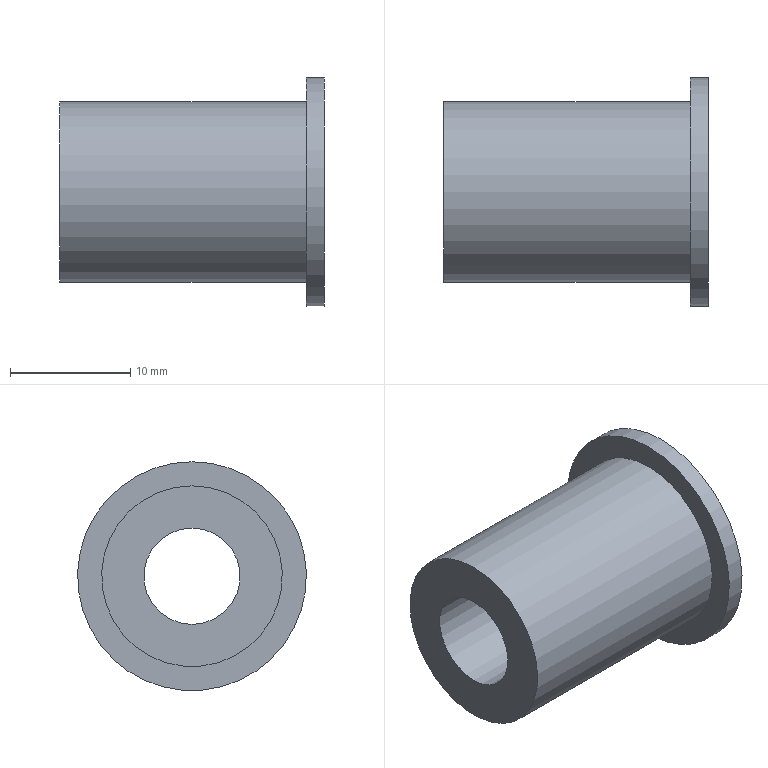Component | NX | HANDLE_BUSHING_2 | 1 solid | 6 faces | box 22 x 19 x 19 mm | volume 2942 mm3 | plane 3 | cylinder 3 | commonest cylinder face diameters 15 x1 19 x1 8 x1
STEP:
#1=CARTESIAN_POINT('',(0.,0.,0.));
#2=DIRECTION('',(0.,0.,1.));
#3=DIRECTION('',(1.,0.,0.));
#4=AXIS2_PLACEMENT_3D('',#1,#2,#3);
#5=CARTESIAN_POINT('',(184.037,-19.732,75.));
#6=VERTEX_POINT('',#5);
#7=CARTESIAN_POINT('',(184.037,-19.732,79.));
#8=DIRECTION('',(1.,0.,0.));
#9=DIRECTION('',(0.,0.,-1.));
#10=AXIS2_PLACEMENT_3D('',#7,#8,#9);
#11=CIRCLE('',#10,4.);
#12=CARTESIAN_POINT('',(184.037,-19.732,79.));
#13=DIRECTION('',(-1.,0.,0.));
#14=DIRECTION('',(0.,0.,1.));
#15=AXIS2_PLACEMENT_3D('',#12,#13,#14);
#16=PLANE('',#15);
#17=CARTESIAN_POINT('',(-4.,0.));
#18=CARTESIAN_POINT('',(-4.,6.928));
#19=CARTESIAN_POINT('',(2.,3.464));
#20=CARTESIAN_POINT('',(8.,0.));
#21=CARTESIAN_POINT('',(2.,-3.464));
#22=CARTESIAN_POINT('',(-4.,-6.928));
#23=CARTESIAN_POINT('',(-4.,0.));
#24=(BOUNDED_CURVE()B_SPLINE_CURVE(2,(#17,#18,#19,#20,#21,#22,#23),.UNSPECIFIED.,.T.,.F.)B_SPLINE_CURVE_WITH_KNOTS((1,2,2,2,2,1),(-2.094,0.,2.094,4.189,6.283,8.378),.UNSPECIFIED.)CURVE()GEOMETRIC_REPRESENTATION_ITEM()RATIONAL_B_SPLINE_CURVE((1.,0.5,1.,0.5,1.,0.5,1.))REPRESENTATION_ITEM(''));
#25=(GEOMETRIC_REPRESENTATION_CONTEXT(2)PARAMETRIC_REPRESENTATION_CONTEXT()REPRESENTATION_CONTEXT('',''));
#26=DEFINITIONAL_REPRESENTATION('',(#24),#25);
#27=PCURVE('',#16,#26);
#28=CARTESIAN_POINT('',(184.037,-19.732,79.));
#29=DIRECTION('',(1.,0.,0.));
#30=DIRECTION('',(0.,0.,-1.));
#31=AXIS2_PLACEMENT_3D('',#28,#29,#30);
#32=CYLINDRICAL_SURFACE('',#31,4.);
#33=CARTESIAN_POINT('',(0.,0.));
#34=DIRECTION('',(1.,0.));
#35=VECTOR('',#34,1.);
#36=LINE('',#33,#35);
#37=(GEOMETRIC_REPRESENTATION_CONTEXT(2)PARAMETRIC_REPRESENTATION_CONTEXT()REPRESENTATION_CONTEXT('',''));
#38=DEFINITIONAL_REPRESENTATION('',(#36),#37);
#39=PCURVE('',#32,#38);
#40=SURFACE_CURVE('',#11,(#27,#39),.PCURVE_S1.);
#41=EDGE_CURVE('',#6,#6,#40,.T.);
#42=ORIENTED_EDGE('',*,*,#41,.T.);
#43=EDGE_LOOP('',(#42));
#44=FACE_BOUND('',#43,.T.);
#45=CARTESIAN_POINT('',(184.037,-19.732,86.5));
#46=VERTEX_POINT('',#45);
#47=CARTESIAN_POINT('',(184.037,-19.732,79.));
#48=DIRECTION('',(1.,0.,0.));
#49=DIRECTION('',(0.,0.,1.));
#50=AXIS2_PLACEMENT_3D('',#47,#48,#49);
#51=CIRCLE('',#50,7.5);
#52=CARTESIAN_POINT('',(7.5,0.));
#53=CARTESIAN_POINT('',(7.5,-12.99));
#54=CARTESIAN_POINT('',(-3.75,-6.495));
#55=CARTESIAN_POINT('',(-15.,-0.));
#56=CARTESIAN_POINT('',(-3.75,6.495));
#57=CARTESIAN_POINT('',(7.5,12.99));
#58=CARTESIAN_POINT('',(7.5,0.));
#59=(BOUNDED_CURVE()B_SPLINE_CURVE(2,(#52,#53,#54,#55,#56,#57,#58),.UNSPECIFIED.,.T.,.F.)B_SPLINE_CURVE_WITH_KNOTS((1,2,2,2,2,1),(-2.094,0.,2.094,4.189,6.283,8.378),.UNSPECIFIED.)CURVE()GEOMETRIC_REPRESENTATION_ITEM()RATIONAL_B_SPLINE_CURVE((1.,0.5,1.,0.5,1.,0.5,1.))REPRESENTATION_ITEM(''));
#60=(GEOMETRIC_REPRESENTATION_CONTEXT(2)PARAMETRIC_REPRESENTATION_CONTEXT()REPRESENTATION_CONTEXT('',''));
#61=DEFINITIONAL_REPRESENTATION('',(#59),#60);
#62=PCURVE('',#16,#61);
#63=CARTESIAN_POINT('',(206.037,-19.732,79.));
#64=DIRECTION('',(-1.,0.,0.));
#65=DIRECTION('',(0.,0.,1.));
#66=AXIS2_PLACEMENT_3D('',#63,#64,#65);
#67=CYLINDRICAL_SURFACE('',#66,7.5);
#68=CARTESIAN_POINT('',(6.283,22.));
#69=DIRECTION('',(-1.,0.));
#70=VECTOR('',#69,1.);
#71=LINE('',#68,#70);
#72=(GEOMETRIC_REPRESENTATION_CONTEXT(2)PARAMETRIC_REPRESENTATION_CONTEXT()REPRESENTATION_CONTEXT('',''));
#73=DEFINITIONAL_REPRESENTATION('',(#71),#72);
#74=PCURVE('',#67,#73);
#75=SURFACE_CURVE('',#51,(#62,#74),.PCURVE_S1.);
#76=EDGE_CURVE('',#46,#46,#75,.T.);
#77=ORIENTED_EDGE('',*,*,#76,.F.);
#78=EDGE_LOOP('',(#77));
#79=FACE_BOUND('',#78,.T.);
#80=ADVANCED_FACE('',(#44,#79),#16,.T.);
#81=CARTESIAN_POINT('',(204.537,-19.732,86.5));
#82=VERTEX_POINT('',#81);
#83=CARTESIAN_POINT('',(204.537,-19.732,79.));
#84=DIRECTION('',(1.,0.,0.));
#85=DIRECTION('',(0.,0.,1.));
#86=AXIS2_PLACEMENT_3D('',#83,#84,#85);
#87=CIRCLE('',#86,7.5);
#88=CARTESIAN_POINT('',(6.283,1.5));
#89=DIRECTION('',(-1.,0.));
#90=VECTOR('',#89,1.);
#91=LINE('',#88,#90);
#92=(GEOMETRIC_REPRESENTATION_CONTEXT(2)PARAMETRIC_REPRESENTATION_CONTEXT()REPRESENTATION_CONTEXT('',''));
#93=DEFINITIONAL_REPRESENTATION('',(#91),#92);
#94=PCURVE('',#67,#93);
#95=CARTESIAN_POINT('',(204.537,-19.732,79.));
#96=DIRECTION('',(-1.,0.,0.));
#97=DIRECTION('',(0.,0.,1.));
#98=AXIS2_PLACEMENT_3D('',#95,#96,#97);
#99=PLANE('',#98);
#100=CARTESIAN_POINT('',(7.5,0.));
#101=CARTESIAN_POINT('',(7.5,-12.99));
#102=CARTESIAN_POINT('',(-3.75,-6.495));
#103=CARTESIAN_POINT('',(-15.,-0.));
#104=CARTESIAN_POINT('',(-3.75,6.495));
#105=CARTESIAN_POINT('',(7.5,12.99));
#106=CARTESIAN_POINT('',(7.5,0.));
#107=(BOUNDED_CURVE()B_SPLINE_CURVE(2,(#100,#101,#102,#103,#104,#105,#106),.UNSPECIFIED.,.T.,.F.)B_SPLINE_CURVE_WITH_KNOTS((1,2,2,2,2,1),(-2.094,0.,2.094,4.189,6.283,8.378),.UNSPECIFIED.)CURVE()GEOMETRIC_REPRESENTATION_ITEM()RATIONAL_B_SPLINE_CURVE((1.,0.5,1.,0.5,1.,0.5,1.))REPRESENTATION_ITEM(''));
#108=(GEOMETRIC_REPRESENTATION_CONTEXT(2)PARAMETRIC_REPRESENTATION_CONTEXT()REPRESENTATION_CONTEXT('',''));
#109=DEFINITIONAL_REPRESENTATION('',(#107),#108);
#110=PCURVE('',#99,#109);
#111=SURFACE_CURVE('',#87,(#94,#110),.PCURVE_S1.);
#112=EDGE_CURVE('',#82,#82,#111,.T.);
#113=ORIENTED_EDGE('',*,*,#112,.F.);
#114=CARTESIAN_POINT('',(204.537,-19.732,86.5));
#115=CARTESIAN_POINT('',(184.037,-19.732,86.5));
#116=B_SPLINE_CURVE_WITH_KNOTS('',1,(#114,#115),.UNSPECIFIED.,.F.,.F.,(2,2),(1.5,22.),.PIECEWISE_BEZIER_KNOTS.);
#117=CARTESIAN_POINT('',(6.283,0.));
#118=DIRECTION('',(0.,1.));
#119=VECTOR('',#118,1.);
#120=LINE('',#117,#119);
#121=(GEOMETRIC_REPRESENTATION_CONTEXT(2)PARAMETRIC_REPRESENTATION_CONTEXT()REPRESENTATION_CONTEXT('',''));
#122=DEFINITIONAL_REPRESENTATION('',(#120),#121);
#123=PCURVE('',#67,#122);
#124=CARTESIAN_POINT('',(0.,0.));
#125=DIRECTION('',(0.,1.));
#126=VECTOR('',#125,1.);
#127=LINE('',#124,#126);
#128=(GEOMETRIC_REPRESENTATION_CONTEXT(2)PARAMETRIC_REPRESENTATION_CONTEXT()REPRESENTATION_CONTEXT('',''));
#129=DEFINITIONAL_REPRESENTATION('',(#127),#128);
#130=PCURVE('',#67,#129);
#131=SEAM_CURVE('',#116,(#123,#130),.PCURVE_S1.);
#132=EDGE_CURVE('',#82,#46,#131,.T.);
#133=ORIENTED_EDGE('',*,*,#132,.T.);
#134=ORIENTED_EDGE('',*,*,#76,.T.);
#135=ORIENTED_EDGE('',*,*,#132,.F.);
#136=EDGE_LOOP('',(#113,#133,#134,#135));
#137=FACE_BOUND('',#136,.T.);
#138=ADVANCED_FACE('',(#137),#67,.T.);
#139=ORIENTED_EDGE('',*,*,#112,.T.);
#140=EDGE_LOOP('',(#139));
#141=FACE_BOUND('',#140,.T.);
#142=CARTESIAN_POINT('',(204.537,-19.732,88.5));
#143=VERTEX_POINT('',#142);
#144=CARTESIAN_POINT('',(204.537,-19.732,79.));
#145=DIRECTION('',(1.,0.,0.));
#146=DIRECTION('',(0.,0.,1.));
#147=AXIS2_PLACEMENT_3D('',#144,#145,#146);
#148=CIRCLE('',#147,9.5);
#149=CARTESIAN_POINT('',(9.5,0.));
#150=CARTESIAN_POINT('',(9.5,-16.454));
#151=CARTESIAN_POINT('',(-4.75,-8.227));
#152=CARTESIAN_POINT('',(-19.,-0.));
#153=CARTESIAN_POINT('',(-4.75,8.227));
#154=CARTESIAN_POINT('',(9.5,16.454));
#155=CARTESIAN_POINT('',(9.5,0.));
#156=(BOUNDED_CURVE()B_SPLINE_CURVE(2,(#149,#150,#151,#152,#153,#154,#155),.UNSPECIFIED.,.T.,.F.)B_SPLINE_CURVE_WITH_KNOTS((1,2,2,2,2,1),(-2.094,0.,2.094,4.189,6.283,8.378),.UNSPECIFIED.)CURVE()GEOMETRIC_REPRESENTATION_ITEM()RATIONAL_B_SPLINE_CURVE((1.,0.5,1.,0.5,1.,0.5,1.))REPRESENTATION_ITEM(''));
#157=(GEOMETRIC_REPRESENTATION_CONTEXT(2)PARAMETRIC_REPRESENTATION_CONTEXT()REPRESENTATION_CONTEXT('',''));
#158=DEFINITIONAL_REPRESENTATION('',(#156),#157);
#159=PCURVE('',#99,#158);
#160=CARTESIAN_POINT('',(206.037,-19.732,79.));
#161=DIRECTION('',(-1.,0.,0.));
#162=DIRECTION('',(0.,0.,1.));
#163=AXIS2_PLACEMENT_3D('',#160,#161,#162);
#164=CYLINDRICAL_SURFACE('',#163,9.5);
#165=CARTESIAN_POINT('',(6.283,1.5));
#166=DIRECTION('',(-1.,0.));
#167=VECTOR('',#166,1.);
#168=LINE('',#165,#167);
#169=(GEOMETRIC_REPRESENTATION_CONTEXT(2)PARAMETRIC_REPRESENTATION_CONTEXT()REPRESENTATION_CONTEXT('',''));
#170=DEFINITIONAL_REPRESENTATION('',(#168),#169);
#171=PCURVE('',#164,#170);
#172=SURFACE_CURVE('',#148,(#159,#171),.PCURVE_S1.);
#173=EDGE_CURVE('',#143,#143,#172,.T.);
#174=ORIENTED_EDGE('',*,*,#173,.F.);
#175=EDGE_LOOP('',(#174));
#176=FACE_BOUND('',#175,.T.);
#177=ADVANCED_FACE('',(#141,#176),#99,.T.);
#178=ORIENTED_EDGE('',*,*,#173,.T.);
#179=CARTESIAN_POINT('',(206.037,-19.732,88.5));
#180=VERTEX_POINT('',#179);
#181=CARTESIAN_POINT('',(206.037,-19.732,88.5));
#182=CARTESIAN_POINT('',(204.537,-19.732,88.5));
#183=B_SPLINE_CURVE_WITH_KNOTS('',1,(#181,#182),.UNSPECIFIED.,.F.,.F.,(2,2),(0.,1.5),.PIECEWISE_BEZIER_KNOTS.);
#184=CARTESIAN_POINT('',(0.,0.));
#185=DIRECTION('',(0.,1.));
#186=VECTOR('',#185,1.);
#187=LINE('',#184,#186);
#188=(GEOMETRIC_REPRESENTATION_CONTEXT(2)PARAMETRIC_REPRESENTATION_CONTEXT()REPRESENTATION_CONTEXT('',''));
#189=DEFINITIONAL_REPRESENTATION('',(#187),#188);
#190=PCURVE('',#164,#189);
#191=CARTESIAN_POINT('',(6.283,0.));
#192=DIRECTION('',(0.,1.));
#193=VECTOR('',#192,1.);
#194=LINE('',#191,#193);
#195=(GEOMETRIC_REPRESENTATION_CONTEXT(2)PARAMETRIC_REPRESENTATION_CONTEXT()REPRESENTATION_CONTEXT('',''));
#196=DEFINITIONAL_REPRESENTATION('',(#194),#195);
#197=PCURVE('',#164,#196);
#198=SEAM_CURVE('',#183,(#190,#197),.PCURVE_S1.);
#199=EDGE_CURVE('',#180,#143,#198,.T.);
#200=ORIENTED_EDGE('',*,*,#199,.F.);
#201=CARTESIAN_POINT('',(206.037,-19.732,79.));
#202=DIRECTION('',(-1.,0.,0.));
#203=DIRECTION('',(0.,0.,1.));
#204=AXIS2_PLACEMENT_3D('',#201,#202,#203);
#205=CIRCLE('',#204,9.5);
#206=CARTESIAN_POINT('',(0.,0.));
#207=DIRECTION('',(1.,0.));
#208=VECTOR('',#207,1.);
#209=LINE('',#206,#208);
#210=(GEOMETRIC_REPRESENTATION_CONTEXT(2)PARAMETRIC_REPRESENTATION_CONTEXT()REPRESENTATION_CONTEXT('',''));
#211=DEFINITIONAL_REPRESENTATION('',(#209),#210);
#212=PCURVE('',#164,#211);
#213=CARTESIAN_POINT('',(206.037,-19.732,79.));
#214=DIRECTION('',(1.,0.,0.));
#215=DIRECTION('',(0.,0.,-1.));
#216=AXIS2_PLACEMENT_3D('',#213,#214,#215);
#217=PLANE('',#216);
#218=CARTESIAN_POINT('',(-9.5,0.));
#219=CARTESIAN_POINT('',(-9.5,16.454));
#220=CARTESIAN_POINT('',(4.75,8.227));
#221=CARTESIAN_POINT('',(19.,0.));
#222=CARTESIAN_POINT('',(4.75,-8.227));
#223=CARTESIAN_POINT('',(-9.5,-16.454));
#224=CARTESIAN_POINT('',(-9.5,0.));
#225=(BOUNDED_CURVE()B_SPLINE_CURVE(2,(#218,#219,#220,#221,#222,#223,#224),.UNSPECIFIED.,.T.,.F.)B_SPLINE_CURVE_WITH_KNOTS((1,2,2,2,2,1),(-2.094,0.,2.094,4.189,6.283,8.378),.UNSPECIFIED.)CURVE()GEOMETRIC_REPRESENTATION_ITEM()RATIONAL_B_SPLINE_CURVE((1.,0.5,1.,0.5,1.,0.5,1.))REPRESENTATION_ITEM(''));
#226=(GEOMETRIC_REPRESENTATION_CONTEXT(2)PARAMETRIC_REPRESENTATION_CONTEXT()REPRESENTATION_CONTEXT('',''));
#227=DEFINITIONAL_REPRESENTATION('',(#225),#226);
#228=PCURVE('',#217,#227);
#229=SURFACE_CURVE('',#205,(#212,#228),.PCURVE_S1.);
#230=EDGE_CURVE('',#180,#180,#229,.T.);
#231=ORIENTED_EDGE('',*,*,#230,.T.);
#232=ORIENTED_EDGE('',*,*,#199,.T.);
#233=EDGE_LOOP('',(#178,#200,#231,#232));
#234=FACE_BOUND('',#233,.T.);
#235=ADVANCED_FACE('',(#234),#164,.T.);
#236=CARTESIAN_POINT('',(206.037,-19.732,75.));
#237=VERTEX_POINT('',#236);
#238=CARTESIAN_POINT('',(206.037,-19.732,79.));
#239=DIRECTION('',(1.,0.,0.));
#240=DIRECTION('',(0.,0.,-1.));
#241=AXIS2_PLACEMENT_3D('',#238,#239,#240);
#242=CIRCLE('',#241,4.);
#243=CARTESIAN_POINT('',(0.,0.));
#244=DIRECTION('',(1.,0.));
#245=AXIS2_PLACEMENT_2D('',#243,#244);
#246=CIRCLE('',#245,4.);
#247=(GEOMETRIC_REPRESENTATION_CONTEXT(2)PARAMETRIC_REPRESENTATION_CONTEXT()REPRESENTATION_CONTEXT('',''));
#248=DEFINITIONAL_REPRESENTATION('',(#246),#247);
#249=PCURVE('',#217,#248);
#250=CARTESIAN_POINT('',(0.,22.));
#251=DIRECTION('',(1.,0.));
#252=VECTOR('',#251,1.);
#253=LINE('',#250,#252);
#254=(GEOMETRIC_REPRESENTATION_CONTEXT(2)PARAMETRIC_REPRESENTATION_CONTEXT()REPRESENTATION_CONTEXT('',''));
#255=DEFINITIONAL_REPRESENTATION('',(#253),#254);
#256=PCURVE('',#32,#255);
#257=SURFACE_CURVE('',#242,(#249,#256),.PCURVE_S1.);
#258=EDGE_CURVE('',#237,#237,#257,.T.);
#259=ORIENTED_EDGE('',*,*,#258,.F.);
#260=EDGE_LOOP('',(#259));
#261=FACE_BOUND('',#260,.T.);
#262=ORIENTED_EDGE('',*,*,#230,.F.);
#263=EDGE_LOOP('',(#262));
#264=FACE_BOUND('',#263,.T.);
#265=ADVANCED_FACE('',(#261,#264),#217,.T.);
#266=ORIENTED_EDGE('',*,*,#258,.F.);
#267=CARTESIAN_POINT('',(184.037,-19.732,75.));
#268=CARTESIAN_POINT('',(206.037,-19.732,75.));
#269=B_SPLINE_CURVE_WITH_KNOTS('',1,(#267,#268),.UNSPECIFIED.,.F.,.F.,(2,2),(0.,22.),.PIECEWISE_BEZIER_KNOTS.);
#270=CARTESIAN_POINT('',(0.,0.));
#271=DIRECTION('',(0.,1.));
#272=VECTOR('',#271,1.);
#273=LINE('',#270,#272);
#274=(GEOMETRIC_REPRESENTATION_CONTEXT(2)PARAMETRIC_REPRESENTATION_CONTEXT()REPRESENTATION_CONTEXT('',''));
#275=DEFINITIONAL_REPRESENTATION('',(#273),#274);
#276=PCURVE('',#32,#275);
#277=CARTESIAN_POINT('',(6.283,0.));
#278=DIRECTION('',(0.,1.));
#279=VECTOR('',#278,1.);
#280=LINE('',#277,#279);
#281=(GEOMETRIC_REPRESENTATION_CONTEXT(2)PARAMETRIC_REPRESENTATION_CONTEXT()REPRESENTATION_CONTEXT('',''));
#282=DEFINITIONAL_REPRESENTATION('',(#280),#281);
#283=PCURVE('',#32,#282);
#284=SEAM_CURVE('',#269,(#276,#283),.PCURVE_S1.);
#285=EDGE_CURVE('',#6,#237,#284,.T.);
#286=ORIENTED_EDGE('',*,*,#285,.F.);
#287=ORIENTED_EDGE('',*,*,#41,.T.);
#288=ORIENTED_EDGE('',*,*,#285,.T.);
#289=EDGE_LOOP('',(#266,#286,#287,#288));
#290=FACE_BOUND('',#289,.F.);
#291=ADVANCED_FACE('',(#290),#32,.F.);
#292=CLOSED_SHELL('',(#80,#138,#177,#235,#265,#291));
#293=MANIFOLD_SOLID_BREP('',#292);
#294=(LENGTH_UNIT()NAMED_UNIT(*)SI_UNIT(.MILLI.,.METRE.));
#295=UNCERTAINTY_MEASURE_WITH_UNIT(LENGTH_MEASURE(0.00001),#294,'','');
#296=(NAMED_UNIT(*)PLANE_ANGLE_UNIT()SI_UNIT($,.RADIAN.));
#297=(NAMED_UNIT(*)SI_UNIT($,.STERADIAN.)SOLID_ANGLE_UNIT());
#298=(GEOMETRIC_REPRESENTATION_CONTEXT(3)GLOBAL_UNCERTAINTY_ASSIGNED_CONTEXT((#295))GLOBAL_UNIT_ASSIGNED_CONTEXT((#294,#296,#297))REPRESENTATION_CONTEXT('',''));
#299=ADVANCED_BREP_SHAPE_REPRESENTATION('',(#4,#293),#298);